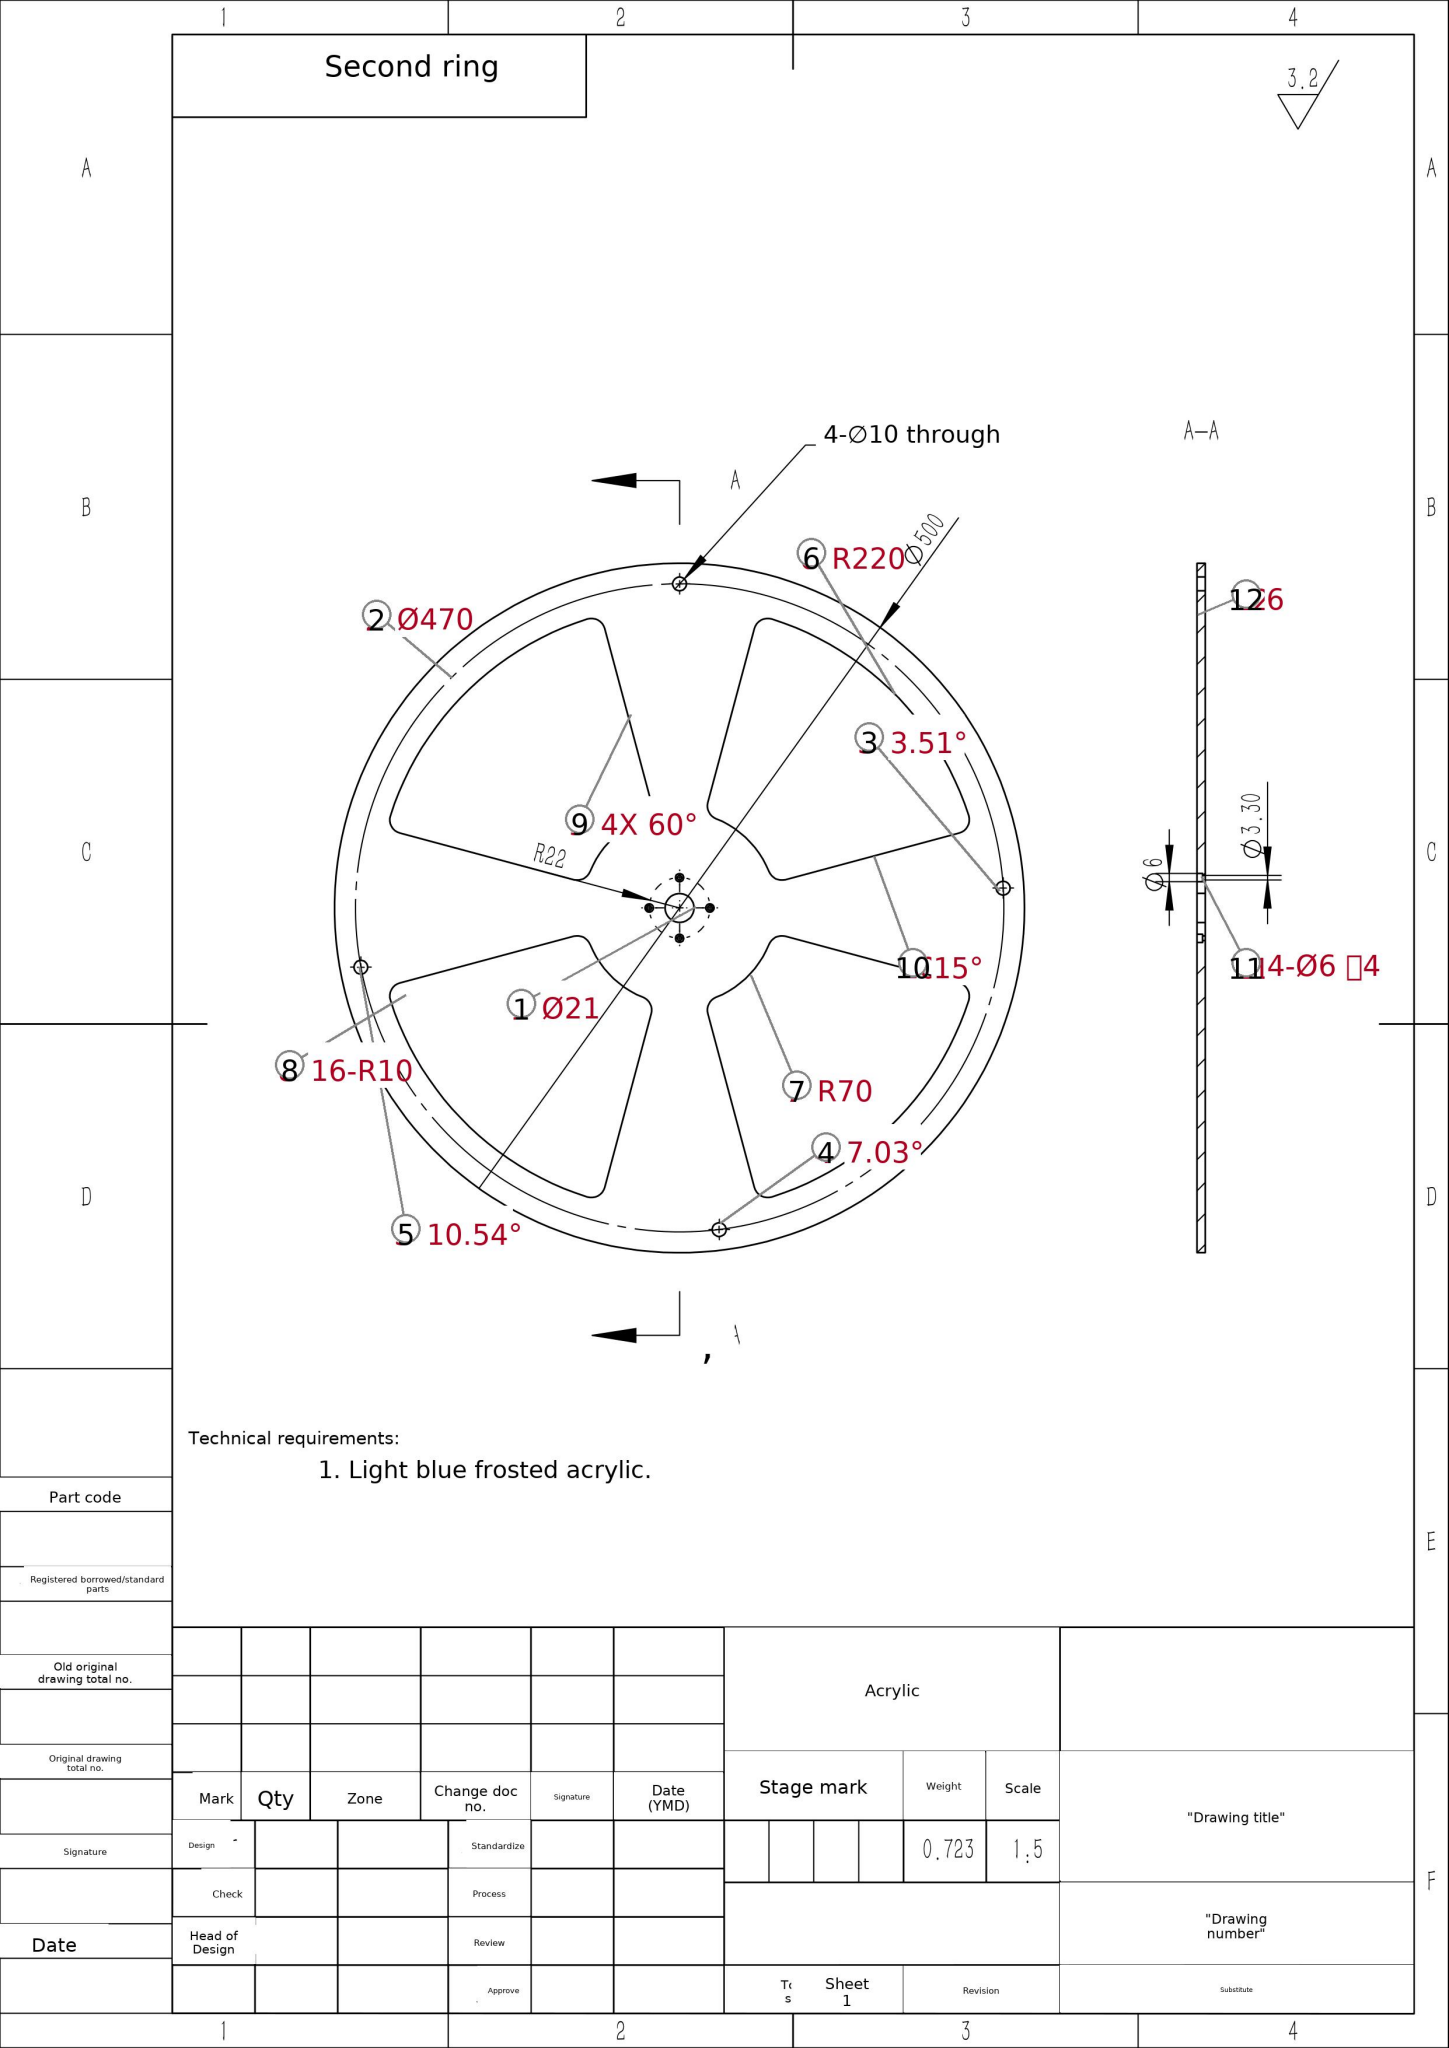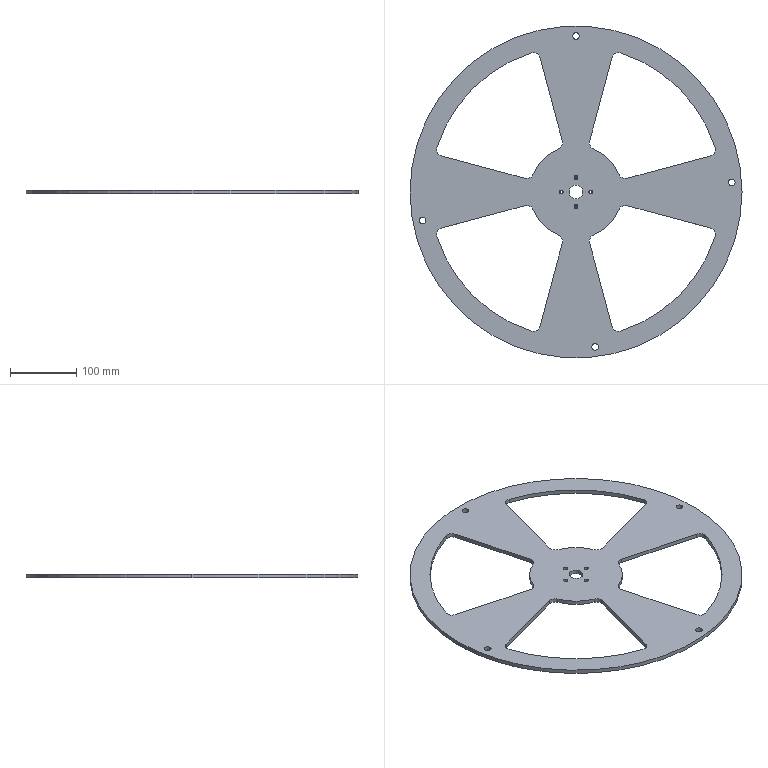Part | SolidWorks | mm | material Acrylic | 1 solid | 70 faces | box 500 x 500 x 6 mm | volume 628926 mm3 | cylinder 56 | plane 14 | commonest cylinder face diameters 20 x20 6 x8 10 x8 3.3 x8 140 x4 440 x4 500 x2 21 x2
build123d program:
from build123d import *

# Parameters (mm, degrees)
SKETCH1_R           = 250
SKETCH1_R_2         = 10.5
BOSS_EXTRUDE1_DEPTH = 3
SKETCH2_R           = 5
CUT_EXTRUDE1_DEPTH  = 10
SKETCH4_R           = 1.65
CUT_EXTRUDE2_DEPTH  = 10
SKETCH5_R           = 3
CUT_EXTRUDE3_DEPTH  = 4
CIRPATTERN1_COUNT   = 4
CUT_EXTRUDE4_DEPTH  = 19
CIRPATTERN2_COUNT   = 4


with BuildPart() as part:
    # Sketch1 → Boss-Extrude1 (new, symmetric)
    with BuildSketch(Plane.XY):
        Circle(SKETCH1_R)
        Circle(SKETCH1_R_2, mode=Mode.SUBTRACT)
    extrude(amount=BOSS_EXTRUDE1_DEPTH, both=True)

    # Sketch2 → Cut-Extrude1 (cut)
    with BuildSketch(Plane.XY.offset(3)):
        with Locations((-231.038, -42.971)):
            Circle(SKETCH2_R)
        with Locations((0, 235)):
            Circle(SKETCH2_R)
        with Locations((234.559, 14.396)):
            Circle(SKETCH2_R)
        with Locations((28.737, -233.236)):
            Circle(SKETCH2_R)
    extrude(amount=-CUT_EXTRUDE1_DEPTH, mode=Mode.SUBTRACT)

    # Sketch4 → Cut-Extrude2 (cut)
    with BuildSketch(Plane.XY.offset(3)):
        with Locations((0, -22)):
            Circle(SKETCH4_R)
    cut_extrude2 = extrude(amount=-CUT_EXTRUDE2_DEPTH, mode=Mode.SUBTRACT)

    # Sketch5 → Cut-Extrude3 (cut)
    with BuildSketch(Plane.XY.offset(3)):
        with Locations((0, -22)):
            Circle(SKETCH5_R)
    cut_extrude3 = extrude(amount=-CUT_EXTRUDE3_DEPTH, mode=Mode.SUBTRACT)

    # CirPattern1: Cut-Extrude2, Cut-Extrude3 ×4 about axis
    cirpattern1_axis = Axis((0, 0, 0), (0, 0, 1))
    add([cut_extrude2.rotate(cirpattern1_axis, i * 360 / CIRPATTERN1_COUNT) for i in range(1, CIRPATTERN1_COUNT)], mode=Mode.SUBTRACT)
    add([cut_extrude3.rotate(cirpattern1_axis, i * 360 / CIRPATTERN1_COUNT) for i in range(1, CIRPATTERN1_COUNT)], mode=Mode.SUBTRACT)

    # Sketch7 → Cut-Extrude4 (cut)
    with BuildSketch(Plane.XY.offset(3)):
        with BuildLine():
            Line((54.29, 202.614), (20.543, 76.668))
            ThreePointArc((20.543, 76.668), (21.246, 69.632), (26.427, 64.82))
            ThreePointArc((26.427, 64.82), (49.497, 49.497), (64.82, 26.427))
            ThreePointArc((64.82, 26.427), (69.632, 21.246), (76.668, 20.543))
            Line((76.668, 20.543), (202.614, 54.29))
            ThreePointArc((202.614, 54.29), (208.803, 59.157), (209.551, 66.995))
            ThreePointArc((209.551, 66.995), (155.563, 155.563), (66.995, 209.551))
            ThreePointArc((66.995, 209.551), (59.157, 208.803), (54.29, 202.614))
        make_face()
    cut_extrude4 = extrude(amount=-CUT_EXTRUDE4_DEPTH, mode=Mode.SUBTRACT)

    # CirPattern2: Cut-Extrude4 ×4 about axis
    cirpattern2_axis = Axis((0, 0, 0), (0, 0, 1))
    for i in range(1, CIRPATTERN2_COUNT):
        add(cut_extrude4.rotate(cirpattern2_axis, i * 360 / CIRPATTERN2_COUNT), mode=Mode.SUBTRACT)


solid = part.part